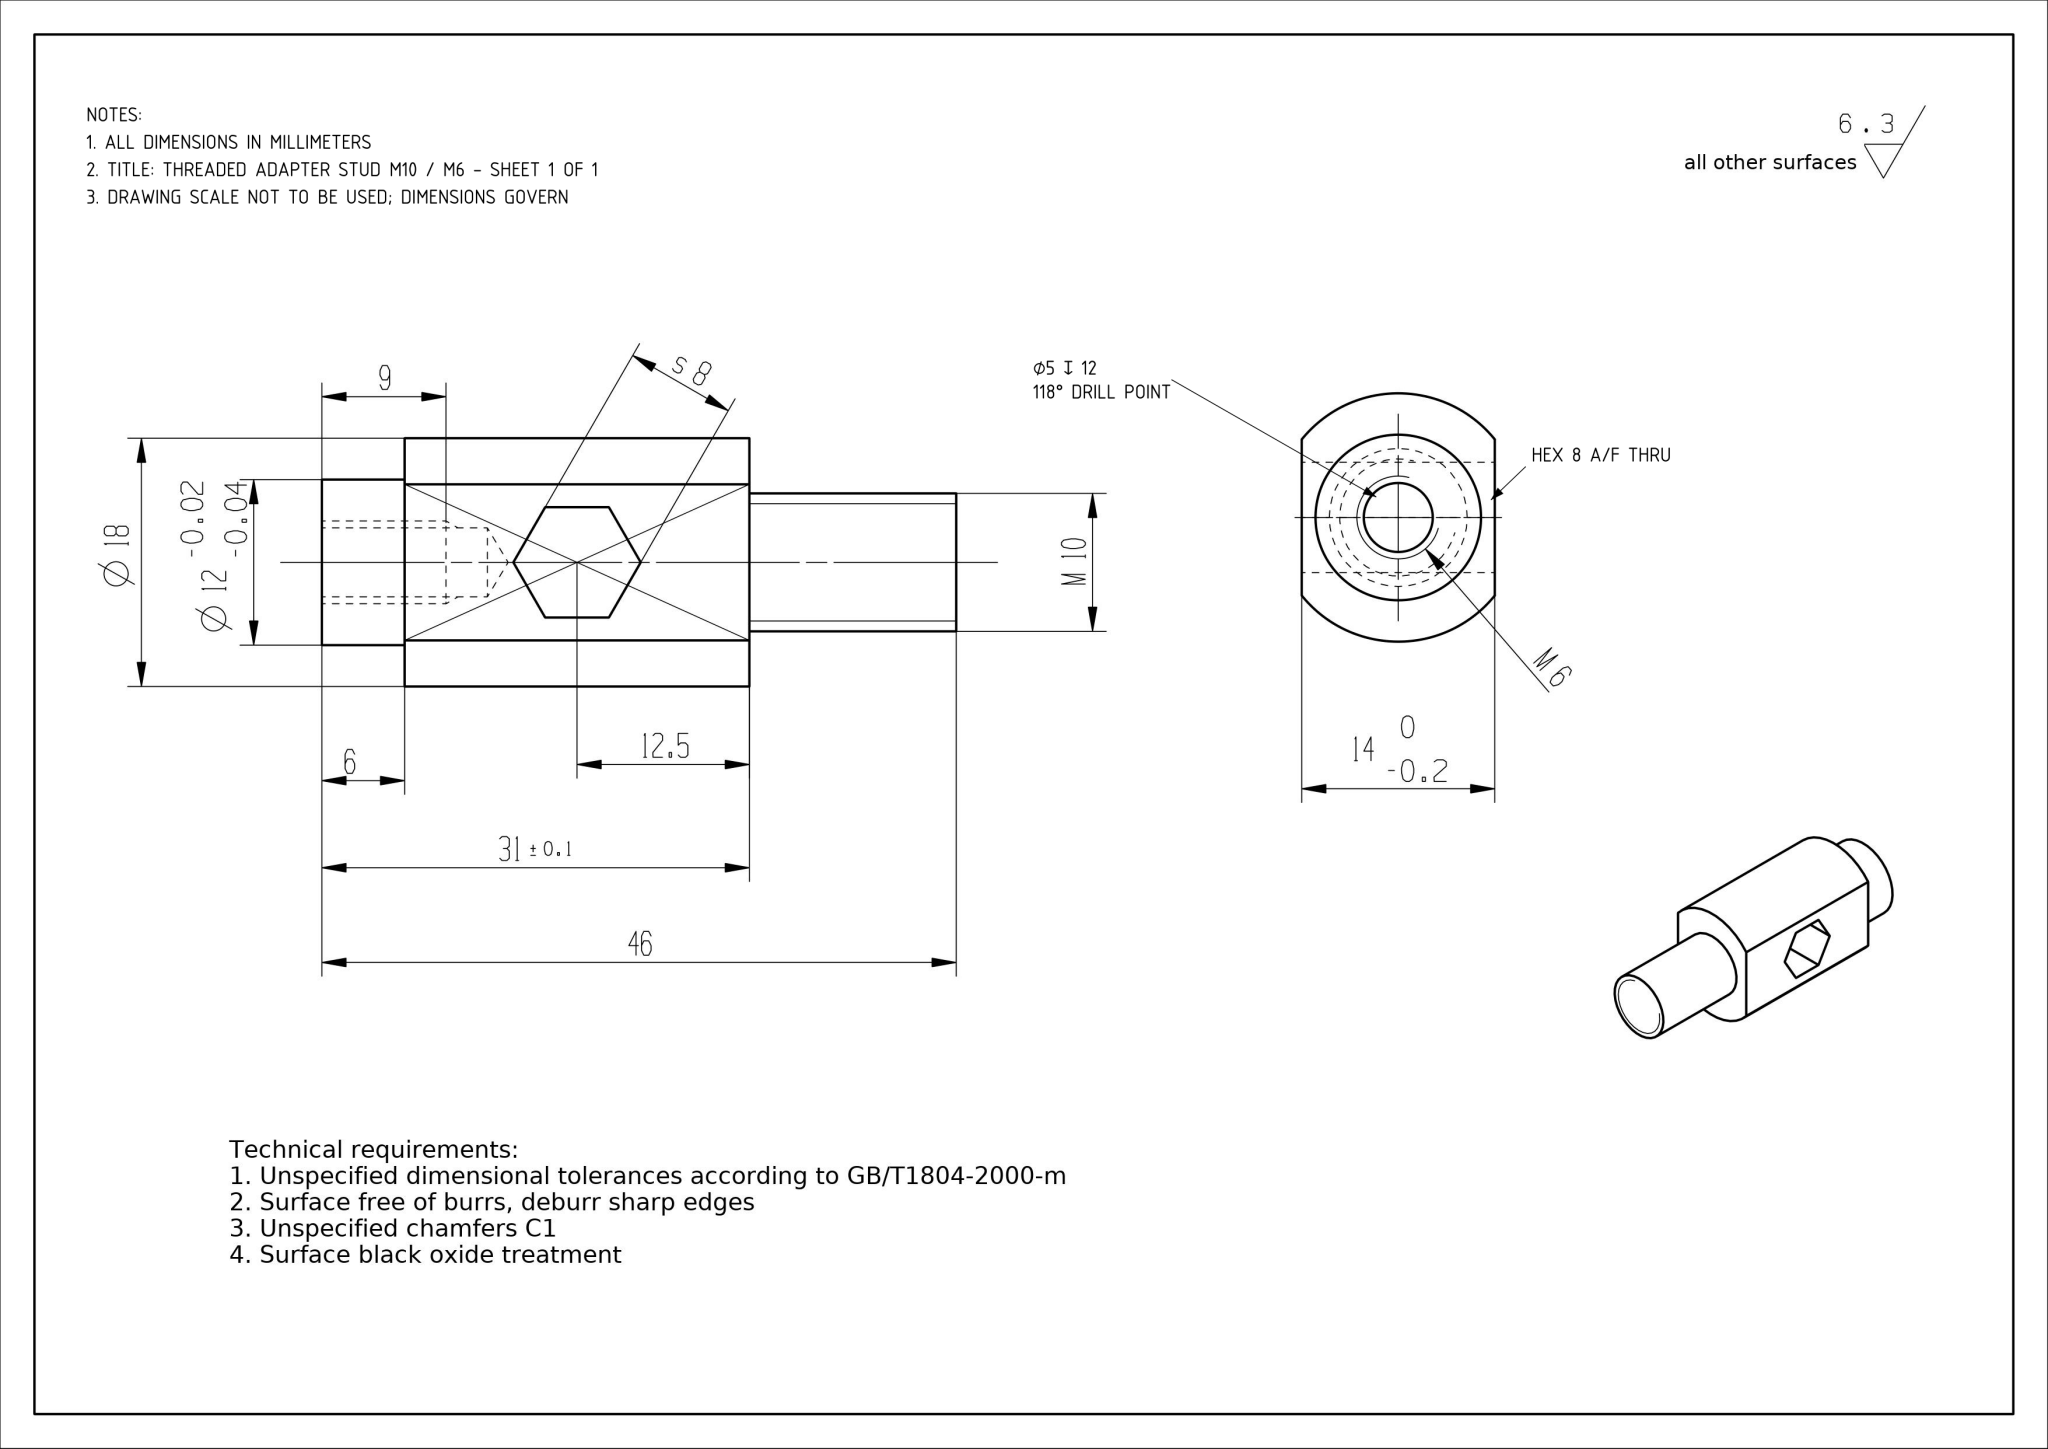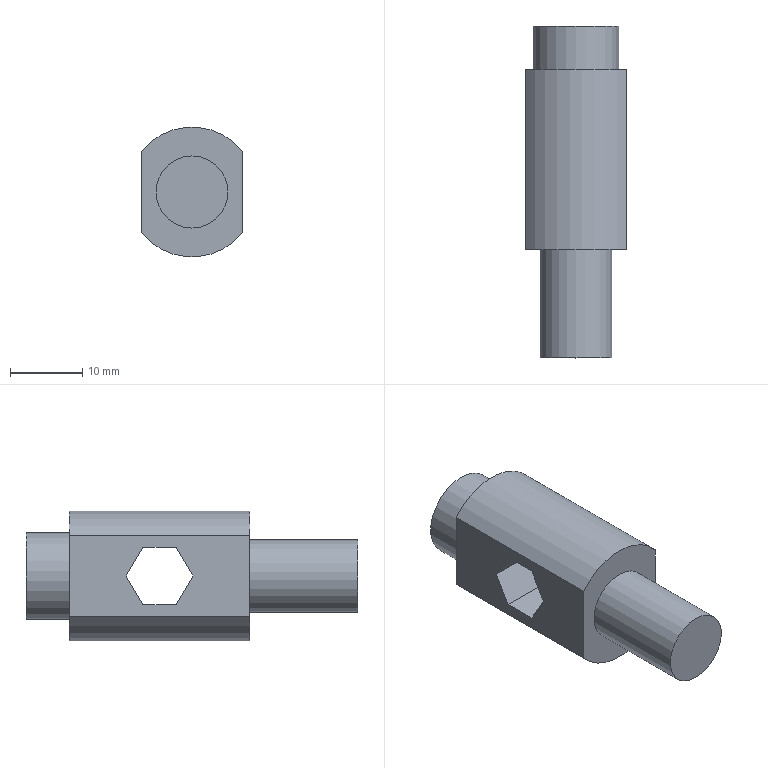Part | NX | mm | 1 solid | 18 faces | box 14 x 46 x 18 mm | volume 6424 mm3 | plane 12 | cylinder 5 | cone 1 | commonest cylinder face diameters 18 x2 12 x1 10 x1 5 x1
STEP:
#1=CARTESIAN_POINT('',(0.,0.,0.));
#2=DIRECTION('',(0.,0.,1.));
#3=DIRECTION('',(1.,0.,0.));
#4=AXIS2_PLACEMENT_3D('',#1,#2,#3);
#5=(LENGTH_UNIT()NAMED_UNIT(*)SI_UNIT(.MILLI.,.METRE.));
#6=UNCERTAINTY_MEASURE_WITH_UNIT(LENGTH_MEASURE(0.00002),#5,'','');
#7=(NAMED_UNIT(*)PLANE_ANGLE_UNIT()SI_UNIT($,.RADIAN.));
#8=PLANE_ANGLE_MEASURE_WITH_UNIT(PLANE_ANGLE_MEASURE(0.01745),#7);
#9=DIMENSIONAL_EXPONENTS(0.,0.,0.,0.,0.,0.,0.);
#10=(CONVERSION_BASED_UNIT('',#8)NAMED_UNIT(#9)PLANE_ANGLE_UNIT());
#11=(NAMED_UNIT(*)SI_UNIT($,.STERADIAN.)SOLID_ANGLE_UNIT());
#12=(GEOMETRIC_REPRESENTATION_CONTEXT(3)GLOBAL_UNCERTAINTY_ASSIGNED_CONTEXT((#6))GLOBAL_UNIT_ASSIGNED_CONTEXT((#5,#10,#11))REPRESENTATION_CONTEXT('',''));
#13=SHAPE_REPRESENTATION('',(#4),#12);
#14=CARTESIAN_POINT('',(7.,25.,5.657));
#15=VERTEX_POINT('',#14);
#16=CARTESIAN_POINT('',(-7.,25.,5.657));
#17=VERTEX_POINT('',#16);
#18=CARTESIAN_POINT('',(0.,25.,0.));
#19=DIRECTION('',(0.,-1.,0.));
#20=DIRECTION('',(0.,-0.,-1.));
#21=AXIS2_PLACEMENT_3D('',#18,#19,#20);
#22=CIRCLE('',#21,9.);
#23=EDGE_CURVE('',#15,#17,#22,.T.);
#24=ORIENTED_EDGE('',*,*,#23,.T.);
#25=CARTESIAN_POINT('',(-7.,0.,5.657));
#26=VERTEX_POINT('',#25);
#27=CARTESIAN_POINT('',(-7.,33.,5.657));
#28=DIRECTION('',(0.,-1.,0.));
#29=VECTOR('',#28,1.);
#30=LINE('',#27,#29);
#31=EDGE_CURVE('',#17,#26,#30,.T.);
#32=ORIENTED_EDGE('',*,*,#31,.T.);
#33=CARTESIAN_POINT('',(7.,0.,5.657));
#34=VERTEX_POINT('',#33);
#35=CARTESIAN_POINT('',(0.,0.,0.));
#36=DIRECTION('',(0.,-1.,0.));
#37=DIRECTION('',(0.,0.,1.));
#38=AXIS2_PLACEMENT_3D('',#35,#36,#37);
#39=CIRCLE('',#38,9.);
#40=EDGE_CURVE('',#34,#26,#39,.T.);
#41=ORIENTED_EDGE('',*,*,#40,.F.);
#42=CARTESIAN_POINT('',(7.,33.,5.657));
#43=DIRECTION('',(0.,1.,-0.));
#44=VECTOR('',#43,1.);
#45=LINE('',#42,#44);
#46=EDGE_CURVE('',#34,#15,#45,.T.);
#47=ORIENTED_EDGE('',*,*,#46,.T.);
#48=EDGE_LOOP('',(#24,#32,#41,#47));
#49=FACE_OUTER_BOUND('',#48,.T.);
#50=CARTESIAN_POINT('',(0.,33.,0.));
#51=DIRECTION('',(0.,-1.,0.));
#52=DIRECTION('',(0.,0.,-1.));
#53=AXIS2_PLACEMENT_3D('',#50,#51,#52);
#54=CYLINDRICAL_SURFACE('',#53,9.);
#55=ADVANCED_FACE('',(#49),#54,.T.);
#56=CARTESIAN_POINT('',(0.,-15.,5.));
#57=VERTEX_POINT('',#56);
#58=CARTESIAN_POINT('',(0.,-15.,0.));
#59=DIRECTION('',(0.,-1.,0.));
#60=DIRECTION('',(0.,0.,1.));
#61=AXIS2_PLACEMENT_3D('',#58,#59,#60);
#62=CIRCLE('',#61,5.);
#63=EDGE_CURVE('',#57,#57,#62,.T.);
#64=ORIENTED_EDGE('',*,*,#63,.T.);
#65=EDGE_LOOP('',(#64));
#66=FACE_OUTER_BOUND('',#65,.T.);
#67=CARTESIAN_POINT('',(0.,-15.,5.));
#68=DIRECTION('',(0.,1.,-0.));
#69=DIRECTION('',(0.,0.,1.));
#70=AXIS2_PLACEMENT_3D('',#67,#68,#69);
#71=PLANE('',#70);
#72=ADVANCED_FACE('',(#66),#71,.F.);
#73=CARTESIAN_POINT('',(0.,31.,-2.5));
#74=VERTEX_POINT('',#73);
#75=CARTESIAN_POINT('',(0.,31.,0.));
#76=DIRECTION('',(0.,-1.,0.));
#77=DIRECTION('',(0.,0.,-1.));
#78=AXIS2_PLACEMENT_3D('',#75,#76,#77);
#79=CIRCLE('',#78,2.5);
#80=EDGE_CURVE('',#74,#74,#79,.T.);
#81=ORIENTED_EDGE('',*,*,#80,.T.);
#82=EDGE_LOOP('',(#81));
#83=FACE_BOUND('',#82,.T.);
#84=CARTESIAN_POINT('',(0.,31.,-6.));
#85=VERTEX_POINT('',#84);
#86=CARTESIAN_POINT('',(0.,31.,0.));
#87=DIRECTION('',(0.,-1.,0.));
#88=DIRECTION('',(0.,-0.,-1.));
#89=AXIS2_PLACEMENT_3D('',#86,#87,#88);
#90=CIRCLE('',#89,6.);
#91=EDGE_CURVE('',#85,#85,#90,.T.);
#92=ORIENTED_EDGE('',*,*,#91,.F.);
#93=EDGE_LOOP('',(#92));
#94=FACE_BOUND('',#93,.T.);
#95=CARTESIAN_POINT('',(0.,31.,0.));
#96=DIRECTION('',(0.,-1.,0.));
#97=DIRECTION('',(0.,-0.,-1.));
#98=AXIS2_PLACEMENT_3D('',#95,#96,#97);
#99=PLANE('',#98);
#100=ADVANCED_FACE('',(#83,#94),#99,.F.);
#101=CARTESIAN_POINT('',(0.,25.,-6.));
#102=VERTEX_POINT('',#101);
#103=CARTESIAN_POINT('',(0.,25.,0.));
#104=DIRECTION('',(0.,-1.,0.));
#105=DIRECTION('',(0.,-0.,-1.));
#106=AXIS2_PLACEMENT_3D('',#103,#104,#105);
#107=CIRCLE('',#106,6.);
#108=EDGE_CURVE('',#102,#102,#107,.T.);
#109=ORIENTED_EDGE('',*,*,#108,.F.);
#110=EDGE_LOOP('',(#109));
#111=FACE_BOUND('',#110,.T.);
#112=ORIENTED_EDGE('',*,*,#91,.T.);
#113=EDGE_LOOP('',(#112));
#114=FACE_BOUND('',#113,.T.);
#115=CARTESIAN_POINT('',(0.,33.,0.));
#116=DIRECTION('',(0.,-1.,0.));
#117=DIRECTION('',(0.,0.,-1.));
#118=AXIS2_PLACEMENT_3D('',#115,#116,#117);
#119=CYLINDRICAL_SURFACE('',#118,6.);
#120=ADVANCED_FACE('',(#111,#114),#119,.T.);
#121=ORIENTED_EDGE('',*,*,#23,.F.);
#122=CARTESIAN_POINT('',(7.,25.,-5.657));
#123=VERTEX_POINT('',#122);
#124=CARTESIAN_POINT('',(7.,25.,11.586));
#125=DIRECTION('',(-0.,-0.,-1.));
#126=VECTOR('',#125,1.);
#127=LINE('',#124,#126);
#128=EDGE_CURVE('',#15,#123,#127,.T.);
#129=ORIENTED_EDGE('',*,*,#128,.T.);
#130=CARTESIAN_POINT('',(-7.,25.,-5.657));
#131=VERTEX_POINT('',#130);
#132=CARTESIAN_POINT('',(0.,25.,0.));
#133=DIRECTION('',(0.,-1.,0.));
#134=DIRECTION('',(0.,-0.,-1.));
#135=AXIS2_PLACEMENT_3D('',#132,#133,#134);
#136=CIRCLE('',#135,9.);
#137=EDGE_CURVE('',#131,#123,#136,.T.);
#138=ORIENTED_EDGE('',*,*,#137,.F.);
#139=CARTESIAN_POINT('',(-7.,25.,-12.137));
#140=DIRECTION('',(0.,0.,1.));
#141=VECTOR('',#140,1.);
#142=LINE('',#139,#141);
#143=EDGE_CURVE('',#131,#17,#142,.T.);
#144=ORIENTED_EDGE('',*,*,#143,.T.);
#145=EDGE_LOOP('',(#121,#129,#138,#144));
#146=FACE_BOUND('',#145,.T.);
#147=ORIENTED_EDGE('',*,*,#108,.T.);
#148=EDGE_LOOP('',(#147));
#149=FACE_BOUND('',#148,.T.);
#150=CARTESIAN_POINT('',(0.,25.,6.));
#151=DIRECTION('',(0.,-1.,0.));
#152=DIRECTION('',(0.,-0.,-1.));
#153=AXIS2_PLACEMENT_3D('',#150,#151,#152);
#154=PLANE('',#153);
#155=ADVANCED_FACE('',(#146,#149),#154,.F.);
#156=CARTESIAN_POINT('',(-7.,-0.,-5.657));
#157=VERTEX_POINT('',#156);
#158=CARTESIAN_POINT('',(7.,-0.,-5.657));
#159=VERTEX_POINT('',#158);
#160=CARTESIAN_POINT('',(0.,0.,0.));
#161=DIRECTION('',(0.,-1.,0.));
#162=DIRECTION('',(0.,0.,1.));
#163=AXIS2_PLACEMENT_3D('',#160,#161,#162);
#164=CIRCLE('',#163,9.);
#165=EDGE_CURVE('',#157,#159,#164,.T.);
#166=ORIENTED_EDGE('',*,*,#165,.F.);
#167=CARTESIAN_POINT('',(-7.,33.,-5.657));
#168=DIRECTION('',(0.,1.,-0.));
#169=VECTOR('',#168,1.);
#170=LINE('',#167,#169);
#171=EDGE_CURVE('',#157,#131,#170,.T.);
#172=ORIENTED_EDGE('',*,*,#171,.T.);
#173=ORIENTED_EDGE('',*,*,#137,.T.);
#174=CARTESIAN_POINT('',(7.,33.,-5.657));
#175=DIRECTION('',(0.,-1.,0.));
#176=VECTOR('',#175,1.);
#177=LINE('',#174,#176);
#178=EDGE_CURVE('',#123,#159,#177,.T.);
#179=ORIENTED_EDGE('',*,*,#178,.T.);
#180=EDGE_LOOP('',(#166,#172,#173,#179));
#181=FACE_OUTER_BOUND('',#180,.T.);
#182=CARTESIAN_POINT('',(0.,33.,0.));
#183=DIRECTION('',(0.,-1.,0.));
#184=DIRECTION('',(0.,0.,-1.));
#185=AXIS2_PLACEMENT_3D('',#182,#183,#184);
#186=CYLINDRICAL_SURFACE('',#185,9.);
#187=ADVANCED_FACE('',(#181),#186,.T.);
#188=CARTESIAN_POINT('',(0.,0.,5.));
#189=VERTEX_POINT('',#188);
#190=CARTESIAN_POINT('',(0.,0.,0.));
#191=DIRECTION('',(0.,-1.,0.));
#192=DIRECTION('',(0.,0.,1.));
#193=AXIS2_PLACEMENT_3D('',#190,#191,#192);
#194=CIRCLE('',#193,5.);
#195=EDGE_CURVE('',#189,#189,#194,.T.);
#196=ORIENTED_EDGE('',*,*,#195,.F.);
#197=EDGE_LOOP('',(#196));
#198=FACE_BOUND('',#197,.T.);
#199=ORIENTED_EDGE('',*,*,#40,.T.);
#200=CARTESIAN_POINT('',(-7.,0.,8.));
#201=DIRECTION('',(-0.,-0.,-1.));
#202=VECTOR('',#201,1.);
#203=LINE('',#200,#202);
#204=EDGE_CURVE('',#26,#157,#203,.T.);
#205=ORIENTED_EDGE('',*,*,#204,.T.);
#206=ORIENTED_EDGE('',*,*,#165,.T.);
#207=CARTESIAN_POINT('',(7.,-0.,8.));
#208=DIRECTION('',(0.,0.,1.));
#209=VECTOR('',#208,1.);
#210=LINE('',#207,#209);
#211=EDGE_CURVE('',#159,#34,#210,.T.);
#212=ORIENTED_EDGE('',*,*,#211,.T.);
#213=EDGE_LOOP('',(#199,#205,#206,#212));
#214=FACE_BOUND('',#213,.T.);
#215=CARTESIAN_POINT('',(0.,0.,8.));
#216=DIRECTION('',(0.,1.,-0.));
#217=DIRECTION('',(0.,0.,1.));
#218=AXIS2_PLACEMENT_3D('',#215,#216,#217);
#219=PLANE('',#218);
#220=ADVANCED_FACE('',(#198,#214),#219,.F.);
#221=ORIENTED_EDGE('',*,*,#63,.F.);
#222=EDGE_LOOP('',(#221));
#223=FACE_BOUND('',#222,.T.);
#224=ORIENTED_EDGE('',*,*,#195,.T.);
#225=EDGE_LOOP('',(#224));
#226=FACE_BOUND('',#225,.T.);
#227=CARTESIAN_POINT('',(0.,33.,0.));
#228=DIRECTION('',(0.,-1.,0.));
#229=DIRECTION('',(0.,0.,-1.));
#230=AXIS2_PLACEMENT_3D('',#227,#228,#229);
#231=CYLINDRICAL_SURFACE('',#230,5.);
#232=ADVANCED_FACE('',(#223,#226),#231,.T.);
#233=CARTESIAN_POINT('',(7.,14.809,-4.));
#234=VERTEX_POINT('',#233);
#235=CARTESIAN_POINT('',(7.,10.191,-4.));
#236=VERTEX_POINT('',#235);
#237=CARTESIAN_POINT('',(7.,25.,-4.));
#238=DIRECTION('',(-0.,-1.,0.));
#239=VECTOR('',#238,1.);
#240=LINE('',#237,#239);
#241=EDGE_CURVE('',#234,#236,#240,.T.);
#242=ORIENTED_EDGE('',*,*,#241,.T.);
#243=CARTESIAN_POINT('',(7.,7.881,0.));
#244=VERTEX_POINT('',#243);
#245=CARTESIAN_POINT('',(7.,7.144,1.277));
#246=DIRECTION('',(0.,-0.5,0.866));
#247=VECTOR('',#246,1.);
#248=LINE('',#245,#247);
#249=EDGE_CURVE('',#236,#244,#248,.T.);
#250=ORIENTED_EDGE('',*,*,#249,.T.);
#251=CARTESIAN_POINT('',(7.,10.191,4.));
#252=VERTEX_POINT('',#251);
#253=CARTESIAN_POINT('',(7.,17.178,16.102));
#254=DIRECTION('',(0.,0.5,0.866));
#255=VECTOR('',#254,1.);
#256=LINE('',#253,#255);
#257=EDGE_CURVE('',#244,#252,#256,.T.);
#258=ORIENTED_EDGE('',*,*,#257,.T.);
#259=CARTESIAN_POINT('',(7.,14.809,4.));
#260=VERTEX_POINT('',#259);
#261=CARTESIAN_POINT('',(7.,25.,4.));
#262=DIRECTION('',(0.,1.,-0.));
#263=VECTOR('',#262,1.);
#264=LINE('',#261,#263);
#265=EDGE_CURVE('',#252,#260,#264,.T.);
#266=ORIENTED_EDGE('',*,*,#265,.T.);
#267=CARTESIAN_POINT('',(7.,17.119,0.));
#268=VERTEX_POINT('',#267);
#269=CARTESIAN_POINT('',(7.,14.072,5.277));
#270=DIRECTION('',(-0.,0.5,-0.866));
#271=VECTOR('',#270,1.);
#272=LINE('',#269,#271);
#273=EDGE_CURVE('',#260,#268,#272,.T.);
#274=ORIENTED_EDGE('',*,*,#273,.T.);
#275=CARTESIAN_POINT('',(7.,24.106,12.102));
#276=DIRECTION('',(-0.,-0.5,-0.866));
#277=VECTOR('',#276,1.);
#278=LINE('',#275,#277);
#279=EDGE_CURVE('',#268,#234,#278,.T.);
#280=ORIENTED_EDGE('',*,*,#279,.T.);
#281=EDGE_LOOP('',(#242,#250,#258,#266,#274,#280));
#282=FACE_BOUND('',#281,.T.);
#283=ORIENTED_EDGE('',*,*,#128,.F.);
#284=ORIENTED_EDGE('',*,*,#46,.F.);
#285=ORIENTED_EDGE('',*,*,#211,.F.);
#286=ORIENTED_EDGE('',*,*,#178,.F.);
#287=EDGE_LOOP('',(#283,#284,#285,#286));
#288=FACE_BOUND('',#287,.T.);
#289=CARTESIAN_POINT('',(7.,25.,11.586));
#290=DIRECTION('',(-1.,0.,0.));
#291=DIRECTION('',(0.,0.,1.));
#292=AXIS2_PLACEMENT_3D('',#289,#290,#291);
#293=PLANE('',#292);
#294=ADVANCED_FACE('',(#282,#288),#293,.F.);
#295=CARTESIAN_POINT('',(-7.,10.191,4.));
#296=VERTEX_POINT('',#295);
#297=CARTESIAN_POINT('',(-7.,7.881,0.));
#298=VERTEX_POINT('',#297);
#299=CARTESIAN_POINT('',(-7.,6.905,-1.69));
#300=DIRECTION('',(-0.,-0.5,-0.866));
#301=VECTOR('',#300,1.);
#302=LINE('',#299,#301);
#303=EDGE_CURVE('',#296,#298,#302,.T.);
#304=ORIENTED_EDGE('',*,*,#303,.T.);
#305=CARTESIAN_POINT('',(-7.,10.191,-4.));
#306=VERTEX_POINT('',#305);
#307=CARTESIAN_POINT('',(-7.,17.416,-16.515));
#308=DIRECTION('',(-0.,0.5,-0.866));
#309=VECTOR('',#308,1.);
#310=LINE('',#307,#309);
#311=EDGE_CURVE('',#298,#306,#310,.T.);
#312=ORIENTED_EDGE('',*,*,#311,.T.);
#313=CARTESIAN_POINT('',(-7.,14.809,-4.));
#314=VERTEX_POINT('',#313);
#315=CARTESIAN_POINT('',(-7.,25.,-4.));
#316=DIRECTION('',(0.,1.,0.));
#317=VECTOR('',#316,1.);
#318=LINE('',#315,#317);
#319=EDGE_CURVE('',#306,#314,#318,.T.);
#320=ORIENTED_EDGE('',*,*,#319,.T.);
#321=CARTESIAN_POINT('',(-7.,17.119,0.));
#322=VERTEX_POINT('',#321);
#323=CARTESIAN_POINT('',(-7.,13.834,-5.69));
#324=DIRECTION('',(0.,0.5,0.866));
#325=VECTOR('',#324,1.);
#326=LINE('',#323,#325);
#327=EDGE_CURVE('',#314,#322,#326,.T.);
#328=ORIENTED_EDGE('',*,*,#327,.T.);
#329=CARTESIAN_POINT('',(-7.,14.809,4.));
#330=VERTEX_POINT('',#329);
#331=CARTESIAN_POINT('',(-7.,24.345,-12.515));
#332=DIRECTION('',(0.,-0.5,0.866));
#333=VECTOR('',#332,1.);
#334=LINE('',#331,#333);
#335=EDGE_CURVE('',#322,#330,#334,.T.);
#336=ORIENTED_EDGE('',*,*,#335,.T.);
#337=CARTESIAN_POINT('',(-7.,25.,4.));
#338=DIRECTION('',(-0.,-1.,0.));
#339=VECTOR('',#338,1.);
#340=LINE('',#337,#339);
#341=EDGE_CURVE('',#330,#296,#340,.T.);
#342=ORIENTED_EDGE('',*,*,#341,.T.);
#343=EDGE_LOOP('',(#304,#312,#320,#328,#336,#342));
#344=FACE_BOUND('',#343,.T.);
#345=ORIENTED_EDGE('',*,*,#143,.F.);
#346=ORIENTED_EDGE('',*,*,#171,.F.);
#347=ORIENTED_EDGE('',*,*,#204,.F.);
#348=ORIENTED_EDGE('',*,*,#31,.F.);
#349=EDGE_LOOP('',(#345,#346,#347,#348));
#350=FACE_BOUND('',#349,.T.);
#351=CARTESIAN_POINT('',(-7.,25.,-12.137));
#352=DIRECTION('',(1.,-0.,-0.));
#353=DIRECTION('',(-0.,0.,-1.));
#354=AXIS2_PLACEMENT_3D('',#351,#352,#353);
#355=PLANE('',#354);
#356=ADVANCED_FACE('',(#344,#350),#355,.F.);
#357=CARTESIAN_POINT('',(0.,19.,-2.5));
#358=VERTEX_POINT('',#357);
#359=CARTESIAN_POINT('',(0.,19.,0.));
#360=DIRECTION('',(0.,1.,-0.));
#361=DIRECTION('',(0.,0.,-1.));
#362=AXIS2_PLACEMENT_3D('',#359,#360,#361);
#363=CIRCLE('',#362,2.5);
#364=EDGE_CURVE('',#358,#358,#363,.T.);
#365=ORIENTED_EDGE('',*,*,#364,.T.);
#366=EDGE_LOOP('',(#365));
#367=FACE_BOUND('',#366,.T.);
#368=CARTESIAN_POINT('',(0.,17.498,0.));
#369=VERTEX_POINT('',#368);
#370=VERTEX_LOOP('',#369);
#371=FACE_BOUND('',#370,.T.);
#372=CARTESIAN_POINT('',(0.,19.,0.));
#373=DIRECTION('',(0.,1.,-0.));
#374=DIRECTION('',(0.,0.,1.));
#375=AXIS2_PLACEMENT_3D('',#372,#373,#374);
#376=CONICAL_SURFACE('',#375,2.5,59.);
#377=ADVANCED_FACE('',(#367,#371),#376,.F.);
#378=ORIENTED_EDGE('',*,*,#364,.F.);
#379=EDGE_LOOP('',(#378));
#380=FACE_BOUND('',#379,.T.);
#381=ORIENTED_EDGE('',*,*,#80,.F.);
#382=EDGE_LOOP('',(#381));
#383=FACE_BOUND('',#382,.T.);
#384=CARTESIAN_POINT('',(0.,31.,0.));
#385=DIRECTION('',(0.,-1.,0.));
#386=DIRECTION('',(0.,0.,-1.));
#387=AXIS2_PLACEMENT_3D('',#384,#385,#386);
#388=CYLINDRICAL_SURFACE('',#387,2.5);
#389=ADVANCED_FACE('',(#380,#383),#388,.F.);
#390=CARTESIAN_POINT('',(-11.,10.191,-4.));
#391=DIRECTION('',(-1.,0.,0.));
#392=VECTOR('',#391,1.);
#393=LINE('',#390,#392);
#394=EDGE_CURVE('',#236,#306,#393,.T.);
#395=ORIENTED_EDGE('',*,*,#394,.T.);
#396=ORIENTED_EDGE('',*,*,#311,.F.);
#397=CARTESIAN_POINT('',(-11.,7.881,0.));
#398=DIRECTION('',(-1.,0.,0.));
#399=VECTOR('',#398,1.);
#400=LINE('',#397,#399);
#401=EDGE_CURVE('',#244,#298,#400,.T.);
#402=ORIENTED_EDGE('',*,*,#401,.F.);
#403=ORIENTED_EDGE('',*,*,#249,.F.);
#404=EDGE_LOOP('',(#395,#396,#402,#403));
#405=FACE_OUTER_BOUND('',#404,.T.);
#406=CARTESIAN_POINT('',(-11.,7.881,0.));
#407=DIRECTION('',(0.,-0.866,-0.5));
#408=DIRECTION('',(0.,0.5,-0.866));
#409=AXIS2_PLACEMENT_3D('',#406,#407,#408);
#410=PLANE('',#409);
#411=ADVANCED_FACE('',(#405),#410,.F.);
#412=CARTESIAN_POINT('',(-11.,14.809,-4.));
#413=DIRECTION('',(-1.,0.,0.));
#414=VECTOR('',#413,1.);
#415=LINE('',#412,#414);
#416=EDGE_CURVE('',#234,#314,#415,.T.);
#417=ORIENTED_EDGE('',*,*,#416,.T.);
#418=ORIENTED_EDGE('',*,*,#319,.F.);
#419=ORIENTED_EDGE('',*,*,#394,.F.);
#420=ORIENTED_EDGE('',*,*,#241,.F.);
#421=EDGE_LOOP('',(#417,#418,#419,#420));
#422=FACE_OUTER_BOUND('',#421,.T.);
#423=CARTESIAN_POINT('',(-11.,10.191,-4.));
#424=DIRECTION('',(0.,0.,-1.));
#425=DIRECTION('',(-1.,0.,0.));
#426=AXIS2_PLACEMENT_3D('',#423,#424,#425);
#427=PLANE('',#426);
#428=ADVANCED_FACE('',(#422),#427,.F.);
#429=CARTESIAN_POINT('',(-11.,17.119,0.));
#430=DIRECTION('',(-1.,0.,0.));
#431=VECTOR('',#430,1.);
#432=LINE('',#429,#431);
#433=EDGE_CURVE('',#268,#322,#432,.T.);
#434=ORIENTED_EDGE('',*,*,#433,.T.);
#435=ORIENTED_EDGE('',*,*,#327,.F.);
#436=ORIENTED_EDGE('',*,*,#416,.F.);
#437=ORIENTED_EDGE('',*,*,#279,.F.);
#438=EDGE_LOOP('',(#434,#435,#436,#437));
#439=FACE_OUTER_BOUND('',#438,.T.);
#440=CARTESIAN_POINT('',(-11.,14.809,-4.));
#441=DIRECTION('',(0.,0.866,-0.5));
#442=DIRECTION('',(0.,0.5,0.866));
#443=AXIS2_PLACEMENT_3D('',#440,#441,#442);
#444=PLANE('',#443);
#445=ADVANCED_FACE('',(#439),#444,.F.);
#446=CARTESIAN_POINT('',(-11.,14.809,4.));
#447=DIRECTION('',(-1.,0.,0.));
#448=VECTOR('',#447,1.);
#449=LINE('',#446,#448);
#450=EDGE_CURVE('',#260,#330,#449,.T.);
#451=ORIENTED_EDGE('',*,*,#450,.T.);
#452=ORIENTED_EDGE('',*,*,#335,.F.);
#453=ORIENTED_EDGE('',*,*,#433,.F.);
#454=ORIENTED_EDGE('',*,*,#273,.F.);
#455=EDGE_LOOP('',(#451,#452,#453,#454));
#456=FACE_OUTER_BOUND('',#455,.T.);
#457=CARTESIAN_POINT('',(-11.,17.119,0.));
#458=DIRECTION('',(0.,0.866,0.5));
#459=DIRECTION('',(0.,-0.5,0.866));
#460=AXIS2_PLACEMENT_3D('',#457,#458,#459);
#461=PLANE('',#460);
#462=ADVANCED_FACE('',(#456),#461,.F.);
#463=CARTESIAN_POINT('',(-11.,10.191,4.));
#464=DIRECTION('',(-1.,0.,0.));
#465=VECTOR('',#464,1.);
#466=LINE('',#463,#465);
#467=EDGE_CURVE('',#252,#296,#466,.T.);
#468=ORIENTED_EDGE('',*,*,#467,.T.);
#469=ORIENTED_EDGE('',*,*,#341,.F.);
#470=ORIENTED_EDGE('',*,*,#450,.F.);
#471=ORIENTED_EDGE('',*,*,#265,.F.);
#472=EDGE_LOOP('',(#468,#469,#470,#471));
#473=FACE_OUTER_BOUND('',#472,.T.);
#474=CARTESIAN_POINT('',(-11.,14.809,4.));
#475=DIRECTION('',(0.,0.,1.));
#476=DIRECTION('',(0.,-1.,0.));
#477=AXIS2_PLACEMENT_3D('',#474,#475,#476);
#478=PLANE('',#477);
#479=ADVANCED_FACE('',(#473),#478,.F.);
#480=ORIENTED_EDGE('',*,*,#401,.T.);
#481=ORIENTED_EDGE('',*,*,#303,.F.);
#482=ORIENTED_EDGE('',*,*,#467,.F.);
#483=ORIENTED_EDGE('',*,*,#257,.F.);
#484=EDGE_LOOP('',(#480,#481,#482,#483));
#485=FACE_OUTER_BOUND('',#484,.T.);
#486=CARTESIAN_POINT('',(-11.,10.191,4.));
#487=DIRECTION('',(0.,-0.866,0.5));
#488=DIRECTION('',(0.,-0.5,-0.866));
#489=AXIS2_PLACEMENT_3D('',#486,#487,#488);
#490=PLANE('',#489);
#491=ADVANCED_FACE('',(#485),#490,.F.);
#492=CLOSED_SHELL('',(#55,#72,#100,#120,#155,#187,#220,#232,#294,#356,#377,#389,#411,#428,#445,#462,#479,#491));
#493=MANIFOLD_SOLID_BREP('',#492);
#494=ADVANCED_BREP_SHAPE_REPRESENTATION('',(#493),#12);
#495=SHAPE_REPRESENTATION_RELATIONSHIP('','',#13,#494);
#496=PRESENTATION_LAYER_ASSIGNMENT('','',(#493));
#497=COLOUR_RGB('',0.298,0.298,0.298);
#498=FILL_AREA_STYLE_COLOUR('',#497);
#499=FILL_AREA_STYLE('',(#498));
#500=SURFACE_STYLE_FILL_AREA(#499);
#501=SURFACE_SIDE_STYLE('',(#500));
#502=SURFACE_STYLE_USAGE(.BOTH.,#501);
#503=PRESENTATION_STYLE_ASSIGNMENT((#502));
#504=STYLED_ITEM('',(#503),#493);
#505=MECHANICAL_DESIGN_GEOMETRIC_PRESENTATION_REPRESENTATION('',(#504),#12);